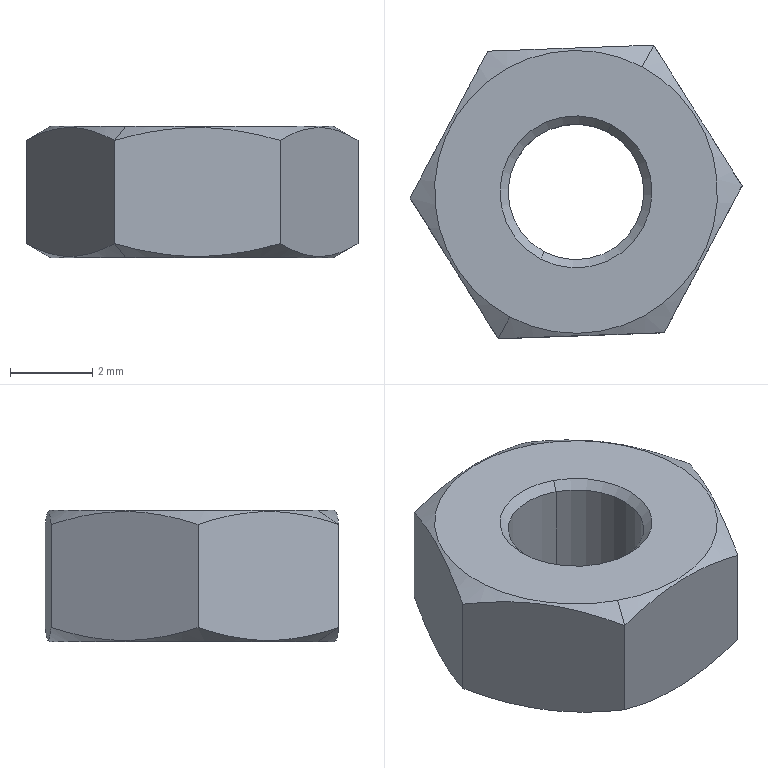Component | SolidWorks | SL010-RightStreamline-1-1_SL010-GB6171-86 M4-1-1 | 1 solid | 18 faces | box 8.08 x 7.14 x 3.2 mm | volume 107 mm3 | cone 8 | plane 8 | cylinder 2 | commonest cylinder face diameters 3.3 x2
STEP:
#1=CARTESIAN_POINT('',(10.403,-4.64,-12.324));
#2=VERTEX_POINT('',#1);
#3=CARTESIAN_POINT('',(10.463,-4.525,-12.324));
#4=VERTEX_POINT('',#3);
#5=CARTESIAN_POINT('',(10.433,-4.583,-12.324));
#6=DIRECTION('',(0.,0.,1.));
#7=DIRECTION('',(-0.4682,-0.8836,0.));
#8=AXIS2_PLACEMENT_3D('',#5,#6,#7);
#9=CIRCLE('',#8,0.06496);
#10=EDGE_CURVE('',#2,#4,#9,.T.);
#11=ORIENTED_EDGE('',*,*,#10,.F.);
#12=CARTESIAN_POINT('',(10.399,-4.647,-12.316));
#13=VERTEX_POINT('',#12);
#14=CARTESIAN_POINT('',(10.399,-4.647,-12.316));
#15=DIRECTION('',(-0.3311,-0.6248,0.7071));
#16=VECTOR('',#15,39.37);
#17=LINE('',#14,#16);
#18=EDGE_CURVE('',#2,#13,#17,.T.);
#19=ORIENTED_EDGE('',*,*,#18,.T.);
#20=CARTESIAN_POINT('',(10.467,-4.518,-12.316));
#21=VERTEX_POINT('',#20);
#22=CARTESIAN_POINT('',(10.433,-4.583,-12.316));
#23=DIRECTION('',(-0.,-0.,-1.));
#24=DIRECTION('',(-0.4682,-0.8836,0.));
#25=AXIS2_PLACEMENT_3D('',#22,#23,#24);
#26=CIRCLE('',#25,0.07283);
#27=EDGE_CURVE('',#21,#13,#26,.T.);
#28=ORIENTED_EDGE('',*,*,#27,.F.);
#29=CARTESIAN_POINT('',(10.467,-4.518,-12.316));
#30=DIRECTION('',(0.3311,0.6248,0.7071));
#31=VECTOR('',#30,39.37);
#32=LINE('',#29,#31);
#33=EDGE_CURVE('',#4,#21,#32,.T.);
#34=ORIENTED_EDGE('',*,*,#33,.F.);
#35=EDGE_LOOP('',(#11,#19,#28,#34));
#36=FACE_OUTER_BOUND('',#35,.T.);
#37=CARTESIAN_POINT('',(10.433,-4.583,-12.316));
#38=DIRECTION('',(0.,0.,1.));
#39=DIRECTION('',(0.4682,0.8836,0.));
#40=AXIS2_PLACEMENT_3D('',#37,#38,#39);
#41=CONICAL_SURFACE('',#40,0.07283,0.7854);
#42=ADVANCED_FACE('',(#36),#41,.F.);
#43=CARTESIAN_POINT('',(10.463,-4.525,-12.434));
#44=VERTEX_POINT('',#43);
#45=CARTESIAN_POINT('',(10.403,-4.64,-12.434));
#46=VERTEX_POINT('',#45);
#47=CARTESIAN_POINT('',(10.433,-4.583,-12.434));
#48=DIRECTION('',(-0.,-0.,-1.));
#49=DIRECTION('',(-0.4682,-0.8836,0.));
#50=AXIS2_PLACEMENT_3D('',#47,#48,#49);
#51=CIRCLE('',#50,0.06496);
#52=EDGE_CURVE('',#44,#46,#51,.T.);
#53=ORIENTED_EDGE('',*,*,#52,.F.);
#54=CARTESIAN_POINT('',(10.467,-4.518,-12.442));
#55=VERTEX_POINT('',#54);
#56=CARTESIAN_POINT('',(10.463,-4.525,-12.434));
#57=DIRECTION('',(0.3311,0.6248,-0.7071));
#58=VECTOR('',#57,39.37);
#59=LINE('',#56,#58);
#60=EDGE_CURVE('',#44,#55,#59,.T.);
#61=ORIENTED_EDGE('',*,*,#60,.T.);
#62=CARTESIAN_POINT('',(10.399,-4.647,-12.442));
#63=VERTEX_POINT('',#62);
#64=CARTESIAN_POINT('',(10.433,-4.583,-12.442));
#65=DIRECTION('',(0.,0.,1.));
#66=DIRECTION('',(-0.4682,-0.8836,0.));
#67=AXIS2_PLACEMENT_3D('',#64,#65,#66);
#68=CIRCLE('',#67,0.07283);
#69=EDGE_CURVE('',#63,#55,#68,.T.);
#70=ORIENTED_EDGE('',*,*,#69,.F.);
#71=CARTESIAN_POINT('',(10.403,-4.64,-12.434));
#72=DIRECTION('',(-0.3311,-0.6248,-0.7071));
#73=VECTOR('',#72,39.37);
#74=LINE('',#71,#73);
#75=EDGE_CURVE('',#46,#63,#74,.T.);
#76=ORIENTED_EDGE('',*,*,#75,.F.);
#77=EDGE_LOOP('',(#53,#61,#70,#76));
#78=FACE_OUTER_BOUND('',#77,.T.);
#79=CARTESIAN_POINT('',(10.433,-4.583,-12.434));
#80=DIRECTION('',(-0.,-0.,-1.));
#81=DIRECTION('',(-0.4682,-0.8836,0.));
#82=AXIS2_PLACEMENT_3D('',#79,#80,#81);
#83=CONICAL_SURFACE('',#82,0.06496,0.7854);
#84=ADVANCED_FACE('',(#78),#83,.F.);
#85=CARTESIAN_POINT('',(10.37,-4.703,-12.442));
#86=VERTEX_POINT('',#85);
#87=CARTESIAN_POINT('',(10.497,-4.463,-12.442));
#88=VERTEX_POINT('',#87);
#89=CARTESIAN_POINT('',(10.433,-4.583,-12.442));
#90=DIRECTION('',(0.,0.,1.));
#91=DIRECTION('',(0.4682,0.8836,0.));
#92=AXIS2_PLACEMENT_3D('',#89,#90,#91);
#93=CIRCLE('',#92,0.1355);
#94=EDGE_CURVE('',#86,#88,#93,.T.);
#95=ORIENTED_EDGE('',*,*,#94,.T.);
#96=CARTESIAN_POINT('',(10.508,-4.442,-12.429));
#97=VERTEX_POINT('',#96);
#98=CARTESIAN_POINT('',(10.497,-4.463,-12.442));
#99=DIRECTION('',(0.4055,0.7652,0.5));
#100=VECTOR('',#99,39.37);
#101=LINE('',#98,#100);
#102=EDGE_CURVE('',#88,#97,#101,.T.);
#103=ORIENTED_EDGE('',*,*,#102,.T.);
#104=CARTESIAN_POINT('',(10.592,-4.577,-12.429));
#105=VERTEX_POINT('',#104);
#106=CARTESIAN_POINT('',(10.508,-4.442,-12.429));
#107=CARTESIAN_POINT('',(10.521,-4.464,-12.436));
#108=CARTESIAN_POINT('',(10.535,-4.487,-12.441));
#109=CARTESIAN_POINT('',(10.557,-4.521,-12.441));
#110=CARTESIAN_POINT('',(10.564,-4.532,-12.44));
#111=CARTESIAN_POINT('',(10.578,-4.555,-12.436));
#112=CARTESIAN_POINT('',(10.585,-4.566,-12.432));
#113=CARTESIAN_POINT('',(10.592,-4.577,-12.429));
#114=B_SPLINE_CURVE_WITH_KNOTS('',3,(#106,#107,#108,#109,#110,#111,#112,#113),.UNSPECIFIED.,.F.,.F.,(4,2,2,4),(0.00000024,0.002041,0.003061,0.004082),.UNSPECIFIED.);
#115=EDGE_CURVE('',#97,#105,#114,.T.);
#116=ORIENTED_EDGE('',*,*,#115,.T.);
#117=CARTESIAN_POINT('',(10.518,-4.718,-12.429));
#118=VERTEX_POINT('',#117);
#119=CARTESIAN_POINT('',(10.592,-4.577,-12.429));
#120=CARTESIAN_POINT('',(10.586,-4.588,-12.432));
#121=CARTESIAN_POINT('',(10.58,-4.6,-12.436));
#122=CARTESIAN_POINT('',(10.567,-4.624,-12.44));
#123=CARTESIAN_POINT('',(10.561,-4.635,-12.441));
#124=CARTESIAN_POINT('',(10.549,-4.659,-12.441));
#125=CARTESIAN_POINT('',(10.542,-4.671,-12.44));
#126=CARTESIAN_POINT('',(10.53,-4.695,-12.436));
#127=CARTESIAN_POINT('',(10.524,-4.706,-12.432));
#128=CARTESIAN_POINT('',(10.518,-4.718,-12.429));
#129=B_SPLINE_CURVE_WITH_KNOTS('',3,(#119,#120,#121,#122,#123,#124,#125,#126,#127,#128),.UNSPECIFIED.,.F.,.F.,(4,2,2,2,4),(0.0036,0.004622,0.005645,0.006667,0.00769),.UNSPECIFIED.);
#130=EDGE_CURVE('',#105,#118,#129,.T.);
#131=ORIENTED_EDGE('',*,*,#130,.T.);
#132=CARTESIAN_POINT('',(10.359,-4.723,-12.429));
#133=VERTEX_POINT('',#132);
#134=CARTESIAN_POINT('',(10.518,-4.718,-12.429));
#135=CARTESIAN_POINT('',(10.492,-4.719,-12.436));
#136=CARTESIAN_POINT('',(10.465,-4.72,-12.441));
#137=CARTESIAN_POINT('',(10.425,-4.721,-12.441));
#138=CARTESIAN_POINT('',(10.411,-4.722,-12.44));
#139=CARTESIAN_POINT('',(10.385,-4.722,-12.436));
#140=CARTESIAN_POINT('',(10.372,-4.723,-12.432));
#141=CARTESIAN_POINT('',(10.359,-4.723,-12.429));
#142=B_SPLINE_CURVE_WITH_KNOTS('',3,(#134,#135,#136,#137,#138,#139,#140,#141),.UNSPECIFIED.,.F.,.F.,(4,2,2,4),(0.00000024,0.002041,0.003061,0.004082),.UNSPECIFIED.);
#143=EDGE_CURVE('',#118,#133,#142,.T.);
#144=ORIENTED_EDGE('',*,*,#143,.T.);
#145=CARTESIAN_POINT('',(10.37,-4.703,-12.442));
#146=DIRECTION('',(-0.4055,-0.7652,0.5));
#147=VECTOR('',#146,39.37);
#148=LINE('',#145,#147);
#149=EDGE_CURVE('',#86,#133,#148,.T.);
#150=ORIENTED_EDGE('',*,*,#149,.F.);
#151=EDGE_LOOP('',(#95,#103,#116,#131,#144,#150));
#152=FACE_OUTER_BOUND('',#151,.T.);
#153=CARTESIAN_POINT('',(10.433,-4.583,-12.442));
#154=DIRECTION('',(0.,0.,1.));
#155=DIRECTION('',(-0.4682,-0.8836,0.));
#156=AXIS2_PLACEMENT_3D('',#153,#154,#155);
#157=CONICAL_SURFACE('',#156,0.1355,1.047);
#158=ADVANCED_FACE('',(#152),#157,.T.);
#159=CARTESIAN_POINT('',(10.497,-4.463,-12.316));
#160=VERTEX_POINT('',#159);
#161=CARTESIAN_POINT('',(10.37,-4.703,-12.316));
#162=VERTEX_POINT('',#161);
#163=CARTESIAN_POINT('',(10.433,-4.583,-12.316));
#164=DIRECTION('',(0.,0.,1.));
#165=DIRECTION('',(0.4682,0.8836,0.));
#166=AXIS2_PLACEMENT_3D('',#163,#164,#165);
#167=CIRCLE('',#166,0.1355);
#168=EDGE_CURVE('',#160,#162,#167,.T.);
#169=ORIENTED_EDGE('',*,*,#168,.F.);
#170=CARTESIAN_POINT('',(10.508,-4.442,-12.33));
#171=VERTEX_POINT('',#170);
#172=CARTESIAN_POINT('',(10.497,-4.463,-12.316));
#173=DIRECTION('',(0.4055,0.7652,-0.5));
#174=VECTOR('',#173,39.37);
#175=LINE('',#172,#174);
#176=EDGE_CURVE('',#160,#171,#175,.T.);
#177=ORIENTED_EDGE('',*,*,#176,.T.);
#178=CARTESIAN_POINT('',(10.349,-4.448,-12.33));
#179=VERTEX_POINT('',#178);
#180=CARTESIAN_POINT('',(10.508,-4.442,-12.33));
#181=CARTESIAN_POINT('',(10.482,-4.443,-12.322));
#182=CARTESIAN_POINT('',(10.455,-4.444,-12.318));
#183=CARTESIAN_POINT('',(10.415,-4.446,-12.318));
#184=CARTESIAN_POINT('',(10.401,-4.446,-12.319));
#185=CARTESIAN_POINT('',(10.375,-4.447,-12.323));
#186=CARTESIAN_POINT('',(10.362,-4.448,-12.326));
#187=CARTESIAN_POINT('',(10.349,-4.448,-12.33));
#188=B_SPLINE_CURVE_WITH_KNOTS('',3,(#180,#181,#182,#183,#184,#185,#186,#187),.UNSPECIFIED.,.F.,.F.,(4,2,2,4),(0.00000024,0.002041,0.003061,0.004082),.UNSPECIFIED.);
#189=EDGE_CURVE('',#171,#179,#188,.T.);
#190=ORIENTED_EDGE('',*,*,#189,.T.);
#191=CARTESIAN_POINT('',(10.274,-4.589,-12.33));
#192=VERTEX_POINT('',#191);
#193=CARTESIAN_POINT('',(10.349,-4.448,-12.33));
#194=CARTESIAN_POINT('',(10.342,-4.459,-12.326));
#195=CARTESIAN_POINT('',(10.336,-4.471,-12.323));
#196=CARTESIAN_POINT('',(10.324,-4.495,-12.319));
#197=CARTESIAN_POINT('',(10.318,-4.506,-12.318));
#198=CARTESIAN_POINT('',(10.305,-4.53,-12.318));
#199=CARTESIAN_POINT('',(10.299,-4.542,-12.319));
#200=CARTESIAN_POINT('',(10.286,-4.566,-12.323));
#201=CARTESIAN_POINT('',(10.28,-4.577,-12.326));
#202=CARTESIAN_POINT('',(10.274,-4.589,-12.33));
#203=B_SPLINE_CURVE_WITH_KNOTS('',3,(#193,#194,#195,#196,#197,#198,#199,#200,#201,#202),.UNSPECIFIED.,.F.,.F.,(4,2,2,2,4),(0.0036,0.004622,0.005645,0.006667,0.00769),.UNSPECIFIED.);
#204=EDGE_CURVE('',#179,#192,#203,.T.);
#205=ORIENTED_EDGE('',*,*,#204,.T.);
#206=CARTESIAN_POINT('',(10.359,-4.723,-12.33));
#207=VERTEX_POINT('',#206);
#208=CARTESIAN_POINT('',(10.274,-4.589,-12.33));
#209=CARTESIAN_POINT('',(10.288,-4.611,-12.322));
#210=CARTESIAN_POINT('',(10.302,-4.633,-12.318));
#211=CARTESIAN_POINT('',(10.323,-4.667,-12.318));
#212=CARTESIAN_POINT('',(10.331,-4.679,-12.319));
#213=CARTESIAN_POINT('',(10.345,-4.701,-12.323));
#214=CARTESIAN_POINT('',(10.352,-4.712,-12.326));
#215=CARTESIAN_POINT('',(10.359,-4.723,-12.33));
#216=B_SPLINE_CURVE_WITH_KNOTS('',3,(#208,#209,#210,#211,#212,#213,#214,#215),.UNSPECIFIED.,.F.,.F.,(4,2,2,4),(0.00000024,0.002041,0.003061,0.004082),.UNSPECIFIED.);
#217=EDGE_CURVE('',#192,#207,#216,.T.);
#218=ORIENTED_EDGE('',*,*,#217,.T.);
#219=CARTESIAN_POINT('',(10.37,-4.703,-12.316));
#220=DIRECTION('',(-0.4055,-0.7652,-0.5));
#221=VECTOR('',#220,39.37);
#222=LINE('',#219,#221);
#223=EDGE_CURVE('',#162,#207,#222,.T.);
#224=ORIENTED_EDGE('',*,*,#223,.F.);
#225=EDGE_LOOP('',(#169,#177,#190,#205,#218,#224));
#226=FACE_OUTER_BOUND('',#225,.T.);
#227=CARTESIAN_POINT('',(10.433,-4.583,-12.316));
#228=DIRECTION('',(-0.,-0.,-1.));
#229=DIRECTION('',(-0.4682,-0.8836,0.));
#230=AXIS2_PLACEMENT_3D('',#227,#228,#229);
#231=CONICAL_SURFACE('',#230,0.1355,1.047);
#232=ADVANCED_FACE('',(#226),#231,.T.);
#233=ORIENTED_EDGE('',*,*,#10,.T.);
#234=CARTESIAN_POINT('',(10.463,-4.525,-12.442));
#235=DIRECTION('',(-0.,-0.,-1.));
#236=VECTOR('',#235,39.37);
#237=LINE('',#234,#236);
#238=EDGE_CURVE('',#4,#44,#237,.T.);
#239=ORIENTED_EDGE('',*,*,#238,.T.);
#240=ORIENTED_EDGE('',*,*,#52,.T.);
#241=CARTESIAN_POINT('',(10.403,-4.64,-12.442));
#242=DIRECTION('',(-0.,-0.,-1.));
#243=VECTOR('',#242,39.37);
#244=LINE('',#241,#243);
#245=EDGE_CURVE('',#2,#46,#244,.T.);
#246=ORIENTED_EDGE('',*,*,#245,.F.);
#247=EDGE_LOOP('',(#233,#239,#240,#246));
#248=FACE_OUTER_BOUND('',#247,.T.);
#249=CARTESIAN_POINT('',(10.433,-4.583,-12.442));
#250=DIRECTION('',(-0.,-0.,-1.));
#251=DIRECTION('',(-0.4682,-0.8836,0.));
#252=AXIS2_PLACEMENT_3D('',#249,#250,#251);
#253=CYLINDRICAL_SURFACE('',#252,0.06496);
#254=ADVANCED_FACE('',(#248),#253,.F.);
#255=ORIENTED_EDGE('',*,*,#143,.F.);
#256=CARTESIAN_POINT('',(10.518,-4.718,-12.33));
#257=VERTEX_POINT('',#256);
#258=CARTESIAN_POINT('',(10.518,-4.718,-12.442));
#259=DIRECTION('',(0.,0.,1.));
#260=VECTOR('',#259,39.37);
#261=LINE('',#258,#260);
#262=EDGE_CURVE('',#118,#257,#261,.T.);
#263=ORIENTED_EDGE('',*,*,#262,.T.);
#264=CARTESIAN_POINT('',(10.359,-4.723,-12.33));
#265=CARTESIAN_POINT('',(10.385,-4.722,-12.322));
#266=CARTESIAN_POINT('',(10.411,-4.722,-12.318));
#267=CARTESIAN_POINT('',(10.451,-4.72,-12.318));
#268=CARTESIAN_POINT('',(10.465,-4.72,-12.319));
#269=CARTESIAN_POINT('',(10.491,-4.719,-12.323));
#270=CARTESIAN_POINT('',(10.505,-4.718,-12.326));
#271=CARTESIAN_POINT('',(10.518,-4.718,-12.33));
#272=B_SPLINE_CURVE_WITH_KNOTS('',3,(#264,#265,#266,#267,#268,#269,#270,#271),.UNSPECIFIED.,.F.,.F.,(4,2,2,4),(0.00000024,0.002041,0.003061,0.004082),.UNSPECIFIED.);
#273=EDGE_CURVE('',#207,#257,#272,.T.);
#274=ORIENTED_EDGE('',*,*,#273,.F.);
#275=CARTESIAN_POINT('',(10.359,-4.723,-12.442));
#276=DIRECTION('',(0.,0.,1.));
#277=VECTOR('',#276,39.37);
#278=LINE('',#275,#277);
#279=EDGE_CURVE('',#133,#207,#278,.T.);
#280=ORIENTED_EDGE('',*,*,#279,.F.);
#281=EDGE_LOOP('',(#255,#263,#274,#280));
#282=FACE_OUTER_BOUND('',#281,.T.);
#283=CARTESIAN_POINT('',(10.518,-4.718,-12.442));
#284=DIRECTION('',(-0.03636,0.9993,-0.));
#285=DIRECTION('',(0.9993,0.03636,-0.));
#286=AXIS2_PLACEMENT_3D('',#283,#284,#285);
#287=PLANE('',#286);
#288=ADVANCED_FACE('',(#282),#287,.F.);
#289=CARTESIAN_POINT('',(10.274,-4.589,-12.429));
#290=VERTEX_POINT('',#289);
#291=CARTESIAN_POINT('',(10.359,-4.723,-12.429));
#292=CARTESIAN_POINT('',(10.345,-4.701,-12.436));
#293=CARTESIAN_POINT('',(10.331,-4.679,-12.441));
#294=CARTESIAN_POINT('',(10.309,-4.645,-12.441));
#295=CARTESIAN_POINT('',(10.302,-4.633,-12.44));
#296=CARTESIAN_POINT('',(10.288,-4.611,-12.436));
#297=CARTESIAN_POINT('',(10.281,-4.6,-12.432));
#298=CARTESIAN_POINT('',(10.274,-4.589,-12.429));
#299=B_SPLINE_CURVE_WITH_KNOTS('',3,(#291,#292,#293,#294,#295,#296,#297,#298),.UNSPECIFIED.,.F.,.F.,(4,2,2,4),(0.00000024,0.002041,0.003061,0.004082),.UNSPECIFIED.);
#300=EDGE_CURVE('',#133,#290,#299,.T.);
#301=ORIENTED_EDGE('',*,*,#300,.F.);
#302=ORIENTED_EDGE('',*,*,#279,.T.);
#303=ORIENTED_EDGE('',*,*,#217,.F.);
#304=CARTESIAN_POINT('',(10.274,-4.589,-12.442));
#305=DIRECTION('',(0.,0.,1.));
#306=VECTOR('',#305,39.37);
#307=LINE('',#304,#306);
#308=EDGE_CURVE('',#290,#192,#307,.T.);
#309=ORIENTED_EDGE('',*,*,#308,.F.);
#310=EDGE_LOOP('',(#301,#302,#303,#309));
#311=FACE_OUTER_BOUND('',#310,.T.);
#312=CARTESIAN_POINT('',(10.359,-4.723,-12.442));
#313=DIRECTION('',(0.8473,0.5312,-0.));
#314=DIRECTION('',(0.5312,-0.8473,0.));
#315=AXIS2_PLACEMENT_3D('',#312,#313,#314);
#316=PLANE('',#315);
#317=ADVANCED_FACE('',(#311),#316,.F.);
#318=CARTESIAN_POINT('',(10.349,-4.448,-12.429));
#319=VERTEX_POINT('',#318);
#320=CARTESIAN_POINT('',(10.274,-4.589,-12.429));
#321=CARTESIAN_POINT('',(10.28,-4.577,-12.432));
#322=CARTESIAN_POINT('',(10.286,-4.566,-12.436));
#323=CARTESIAN_POINT('',(10.299,-4.542,-12.44));
#324=CARTESIAN_POINT('',(10.305,-4.53,-12.441));
#325=CARTESIAN_POINT('',(10.318,-4.506,-12.441));
#326=CARTESIAN_POINT('',(10.324,-4.495,-12.44));
#327=CARTESIAN_POINT('',(10.336,-4.471,-12.436));
#328=CARTESIAN_POINT('',(10.342,-4.459,-12.432));
#329=CARTESIAN_POINT('',(10.349,-4.448,-12.429));
#330=B_SPLINE_CURVE_WITH_KNOTS('',3,(#320,#321,#322,#323,#324,#325,#326,#327,#328,#329),.UNSPECIFIED.,.F.,.F.,(4,2,2,2,4),(0.001487,0.002507,0.003526,0.004546,0.005566),.UNSPECIFIED.);
#331=EDGE_CURVE('',#290,#319,#330,.T.);
#332=ORIENTED_EDGE('',*,*,#331,.F.);
#333=ORIENTED_EDGE('',*,*,#308,.T.);
#334=ORIENTED_EDGE('',*,*,#204,.F.);
#335=CARTESIAN_POINT('',(10.349,-4.448,-12.442));
#336=DIRECTION('',(0.,0.,1.));
#337=VECTOR('',#336,39.37);
#338=LINE('',#335,#337);
#339=EDGE_CURVE('',#319,#179,#338,.T.);
#340=ORIENTED_EDGE('',*,*,#339,.F.);
#341=EDGE_LOOP('',(#332,#333,#334,#340));
#342=FACE_OUTER_BOUND('',#341,.T.);
#343=CARTESIAN_POINT('',(10.274,-4.589,-12.442));
#344=DIRECTION('',(0.8836,-0.4682,0.));
#345=DIRECTION('',(0.,0.,1.));
#346=AXIS2_PLACEMENT_3D('',#343,#344,#345);
#347=PLANE('',#346);
#348=ADVANCED_FACE('',(#342),#347,.F.);
#349=CARTESIAN_POINT('',(10.349,-4.448,-12.429));
#350=CARTESIAN_POINT('',(10.375,-4.447,-12.436));
#351=CARTESIAN_POINT('',(10.401,-4.446,-12.441));
#352=CARTESIAN_POINT('',(10.441,-4.445,-12.441));
#353=CARTESIAN_POINT('',(10.455,-4.444,-12.44));
#354=CARTESIAN_POINT('',(10.481,-4.443,-12.436));
#355=CARTESIAN_POINT('',(10.495,-4.443,-12.432));
#356=CARTESIAN_POINT('',(10.508,-4.442,-12.429));
#357=B_SPLINE_CURVE_WITH_KNOTS('',3,(#349,#350,#351,#352,#353,#354,#355,#356),.UNSPECIFIED.,.F.,.F.,(4,2,2,4),(0.00000024,0.002041,0.003061,0.004082),.UNSPECIFIED.);
#358=EDGE_CURVE('',#319,#97,#357,.T.);
#359=ORIENTED_EDGE('',*,*,#358,.F.);
#360=ORIENTED_EDGE('',*,*,#339,.T.);
#361=ORIENTED_EDGE('',*,*,#189,.F.);
#362=CARTESIAN_POINT('',(10.508,-4.442,-12.442));
#363=DIRECTION('',(0.,0.,1.));
#364=VECTOR('',#363,39.37);
#365=LINE('',#362,#364);
#366=EDGE_CURVE('',#97,#171,#365,.T.);
#367=ORIENTED_EDGE('',*,*,#366,.F.);
#368=EDGE_LOOP('',(#359,#360,#361,#367));
#369=FACE_OUTER_BOUND('',#368,.T.);
#370=CARTESIAN_POINT('',(10.349,-4.448,-12.442));
#371=DIRECTION('',(0.03636,-0.9993,0.));
#372=DIRECTION('',(-0.9993,-0.03636,0.));
#373=AXIS2_PLACEMENT_3D('',#370,#371,#372);
#374=PLANE('',#373);
#375=ADVANCED_FACE('',(#369),#374,.F.);
#376=ORIENTED_EDGE('',*,*,#115,.F.);
#377=ORIENTED_EDGE('',*,*,#366,.T.);
#378=CARTESIAN_POINT('',(10.592,-4.577,-12.33));
#379=VERTEX_POINT('',#378);
#380=CARTESIAN_POINT('',(10.592,-4.577,-12.33));
#381=CARTESIAN_POINT('',(10.578,-4.555,-12.322));
#382=CARTESIAN_POINT('',(10.564,-4.533,-12.318));
#383=CARTESIAN_POINT('',(10.543,-4.498,-12.318));
#384=CARTESIAN_POINT('',(10.536,-4.487,-12.319));
#385=CARTESIAN_POINT('',(10.521,-4.464,-12.323));
#386=CARTESIAN_POINT('',(10.514,-4.453,-12.326));
#387=CARTESIAN_POINT('',(10.508,-4.442,-12.33));
#388=B_SPLINE_CURVE_WITH_KNOTS('',3,(#380,#381,#382,#383,#384,#385,#386,#387),.UNSPECIFIED.,.F.,.F.,(4,2,2,4),(0.00000024,0.002041,0.003061,0.004082),.UNSPECIFIED.);
#389=EDGE_CURVE('',#379,#171,#388,.T.);
#390=ORIENTED_EDGE('',*,*,#389,.F.);
#391=CARTESIAN_POINT('',(10.592,-4.577,-12.442));
#392=DIRECTION('',(0.,0.,1.));
#393=VECTOR('',#392,39.37);
#394=LINE('',#391,#393);
#395=EDGE_CURVE('',#105,#379,#394,.T.);
#396=ORIENTED_EDGE('',*,*,#395,.F.);
#397=EDGE_LOOP('',(#376,#377,#390,#396));
#398=FACE_OUTER_BOUND('',#397,.T.);
#399=CARTESIAN_POINT('',(10.508,-4.442,-12.442));
#400=DIRECTION('',(-0.8473,-0.5312,0.));
#401=DIRECTION('',(-0.5312,0.8473,-0.));
#402=AXIS2_PLACEMENT_3D('',#399,#400,#401);
#403=PLANE('',#402);
#404=ADVANCED_FACE('',(#398),#403,.F.);
#405=ORIENTED_EDGE('',*,*,#130,.F.);
#406=ORIENTED_EDGE('',*,*,#395,.T.);
#407=CARTESIAN_POINT('',(10.518,-4.718,-12.33));
#408=CARTESIAN_POINT('',(10.524,-4.706,-12.326));
#409=CARTESIAN_POINT('',(10.53,-4.695,-12.323));
#410=CARTESIAN_POINT('',(10.542,-4.671,-12.319));
#411=CARTESIAN_POINT('',(10.549,-4.659,-12.318));
#412=CARTESIAN_POINT('',(10.561,-4.635,-12.318));
#413=CARTESIAN_POINT('',(10.567,-4.624,-12.319));
#414=CARTESIAN_POINT('',(10.58,-4.6,-12.323));
#415=CARTESIAN_POINT('',(10.586,-4.588,-12.326));
#416=CARTESIAN_POINT('',(10.592,-4.577,-12.33));
#417=B_SPLINE_CURVE_WITH_KNOTS('',3,(#407,#408,#409,#410,#411,#412,#413,#414,#415,#416),.UNSPECIFIED.,.F.,.F.,(4,2,2,2,4),(0.001487,0.002507,0.003526,0.004546,0.005566),.UNSPECIFIED.);
#418=EDGE_CURVE('',#257,#379,#417,.T.);
#419=ORIENTED_EDGE('',*,*,#418,.F.);
#420=ORIENTED_EDGE('',*,*,#262,.F.);
#421=EDGE_LOOP('',(#405,#406,#419,#420));
#422=FACE_OUTER_BOUND('',#421,.T.);
#423=CARTESIAN_POINT('',(10.592,-4.577,-12.442));
#424=DIRECTION('',(-0.8836,0.4682,-0.));
#425=DIRECTION('',(-0.,-0.,-1.));
#426=AXIS2_PLACEMENT_3D('',#423,#424,#425);
#427=PLANE('',#426);
#428=ADVANCED_FACE('',(#422),#427,.F.);
#429=ORIENTED_EDGE('',*,*,#69,.T.);
#430=CARTESIAN_POINT('',(10.433,-4.583,-12.442));
#431=DIRECTION('',(0.,0.,1.));
#432=DIRECTION('',(-0.4682,-0.8836,0.));
#433=AXIS2_PLACEMENT_3D('',#430,#431,#432);
#434=CIRCLE('',#433,0.07283);
#435=EDGE_CURVE('',#55,#63,#434,.T.);
#436=ORIENTED_EDGE('',*,*,#435,.T.);
#437=EDGE_LOOP('',(#429,#436));
#438=FACE_BOUND('',#437,.T.);
#439=ORIENTED_EDGE('',*,*,#94,.F.);
#440=CARTESIAN_POINT('',(10.433,-4.583,-12.442));
#441=DIRECTION('',(0.,0.,1.));
#442=DIRECTION('',(0.4682,0.8836,0.));
#443=AXIS2_PLACEMENT_3D('',#440,#441,#442);
#444=CIRCLE('',#443,0.1355);
#445=EDGE_CURVE('',#88,#86,#444,.T.);
#446=ORIENTED_EDGE('',*,*,#445,.F.);
#447=EDGE_LOOP('',(#439,#446));
#448=FACE_OUTER_BOUND('',#447,.T.);
#449=CARTESIAN_POINT('',(10.359,-4.723,-12.442));
#450=DIRECTION('',(-0.,-0.,-1.));
#451=DIRECTION('',(-0.4682,-0.8836,0.));
#452=AXIS2_PLACEMENT_3D('',#449,#450,#451);
#453=PLANE('',#452);
#454=ADVANCED_FACE('',(#438,#448),#453,.T.);
#455=ORIENTED_EDGE('',*,*,#27,.T.);
#456=CARTESIAN_POINT('',(10.433,-4.583,-12.316));
#457=DIRECTION('',(-0.,-0.,-1.));
#458=DIRECTION('',(-0.4682,-0.8836,0.));
#459=AXIS2_PLACEMENT_3D('',#456,#457,#458);
#460=CIRCLE('',#459,0.07283);
#461=EDGE_CURVE('',#13,#21,#460,.T.);
#462=ORIENTED_EDGE('',*,*,#461,.T.);
#463=EDGE_LOOP('',(#455,#462));
#464=FACE_BOUND('',#463,.T.);
#465=CARTESIAN_POINT('',(10.433,-4.583,-12.316));
#466=DIRECTION('',(0.,0.,1.));
#467=DIRECTION('',(0.4682,0.8836,0.));
#468=AXIS2_PLACEMENT_3D('',#465,#466,#467);
#469=CIRCLE('',#468,0.1355);
#470=EDGE_CURVE('',#162,#160,#469,.T.);
#471=ORIENTED_EDGE('',*,*,#470,.T.);
#472=ORIENTED_EDGE('',*,*,#168,.T.);
#473=EDGE_LOOP('',(#471,#472));
#474=FACE_OUTER_BOUND('',#473,.T.);
#475=CARTESIAN_POINT('',(10.359,-4.723,-12.316));
#476=DIRECTION('',(-0.,-0.,-1.));
#477=DIRECTION('',(-0.4682,-0.8836,0.));
#478=AXIS2_PLACEMENT_3D('',#475,#476,#477);
#479=PLANE('',#478);
#480=ADVANCED_FACE('',(#464,#474),#479,.F.);
#481=ORIENTED_EDGE('',*,*,#238,.F.);
#482=CARTESIAN_POINT('',(10.433,-4.583,-12.324));
#483=DIRECTION('',(0.,0.,1.));
#484=DIRECTION('',(-0.4682,-0.8836,0.));
#485=AXIS2_PLACEMENT_3D('',#482,#483,#484);
#486=CIRCLE('',#485,0.06496);
#487=EDGE_CURVE('',#4,#2,#486,.T.);
#488=ORIENTED_EDGE('',*,*,#487,.T.);
#489=ORIENTED_EDGE('',*,*,#245,.T.);
#490=CARTESIAN_POINT('',(10.433,-4.583,-12.434));
#491=DIRECTION('',(-0.,-0.,-1.));
#492=DIRECTION('',(-0.4682,-0.8836,0.));
#493=AXIS2_PLACEMENT_3D('',#490,#491,#492);
#494=CIRCLE('',#493,0.06496);
#495=EDGE_CURVE('',#46,#44,#494,.T.);
#496=ORIENTED_EDGE('',*,*,#495,.T.);
#497=EDGE_LOOP('',(#481,#488,#489,#496));
#498=FACE_OUTER_BOUND('',#497,.T.);
#499=CARTESIAN_POINT('',(10.433,-4.583,-12.442));
#500=DIRECTION('',(-0.,-0.,-1.));
#501=DIRECTION('',(-0.4682,-0.8836,0.));
#502=AXIS2_PLACEMENT_3D('',#499,#500,#501);
#503=CYLINDRICAL_SURFACE('',#502,0.06496);
#504=ADVANCED_FACE('',(#498),#503,.F.);
#505=ORIENTED_EDGE('',*,*,#176,.F.);
#506=ORIENTED_EDGE('',*,*,#470,.F.);
#507=ORIENTED_EDGE('',*,*,#223,.T.);
#508=ORIENTED_EDGE('',*,*,#273,.T.);
#509=ORIENTED_EDGE('',*,*,#418,.T.);
#510=ORIENTED_EDGE('',*,*,#389,.T.);
#511=EDGE_LOOP('',(#505,#506,#507,#508,#509,#510));
#512=FACE_OUTER_BOUND('',#511,.T.);
#513=CARTESIAN_POINT('',(10.433,-4.583,-12.316));
#514=DIRECTION('',(-0.,-0.,-1.));
#515=DIRECTION('',(-0.4682,-0.8836,0.));
#516=AXIS2_PLACEMENT_3D('',#513,#514,#515);
#517=CONICAL_SURFACE('',#516,0.1355,1.047);
#518=ADVANCED_FACE('',(#512),#517,.T.);
#519=ORIENTED_EDGE('',*,*,#102,.F.);
#520=ORIENTED_EDGE('',*,*,#445,.T.);
#521=ORIENTED_EDGE('',*,*,#149,.T.);
#522=ORIENTED_EDGE('',*,*,#300,.T.);
#523=ORIENTED_EDGE('',*,*,#331,.T.);
#524=ORIENTED_EDGE('',*,*,#358,.T.);
#525=EDGE_LOOP('',(#519,#520,#521,#522,#523,#524));
#526=FACE_OUTER_BOUND('',#525,.T.);
#527=CARTESIAN_POINT('',(10.433,-4.583,-12.442));
#528=DIRECTION('',(0.,0.,1.));
#529=DIRECTION('',(-0.4682,-0.8836,0.));
#530=AXIS2_PLACEMENT_3D('',#527,#528,#529);
#531=CONICAL_SURFACE('',#530,0.1355,1.047);
#532=ADVANCED_FACE('',(#526),#531,.T.);
#533=ORIENTED_EDGE('',*,*,#60,.F.);
#534=ORIENTED_EDGE('',*,*,#495,.F.);
#535=ORIENTED_EDGE('',*,*,#75,.T.);
#536=ORIENTED_EDGE('',*,*,#435,.F.);
#537=EDGE_LOOP('',(#533,#534,#535,#536));
#538=FACE_OUTER_BOUND('',#537,.T.);
#539=CARTESIAN_POINT('',(10.433,-4.583,-12.434));
#540=DIRECTION('',(-0.,-0.,-1.));
#541=DIRECTION('',(-0.4682,-0.8836,0.));
#542=AXIS2_PLACEMENT_3D('',#539,#540,#541);
#543=CONICAL_SURFACE('',#542,0.06496,0.7854);
#544=ADVANCED_FACE('',(#538),#543,.F.);
#545=ORIENTED_EDGE('',*,*,#18,.F.);
#546=ORIENTED_EDGE('',*,*,#487,.F.);
#547=ORIENTED_EDGE('',*,*,#33,.T.);
#548=ORIENTED_EDGE('',*,*,#461,.F.);
#549=EDGE_LOOP('',(#545,#546,#547,#548));
#550=FACE_OUTER_BOUND('',#549,.T.);
#551=CARTESIAN_POINT('',(10.433,-4.583,-12.316));
#552=DIRECTION('',(0.,0.,1.));
#553=DIRECTION('',(0.4682,0.8836,0.));
#554=AXIS2_PLACEMENT_3D('',#551,#552,#553);
#555=CONICAL_SURFACE('',#554,0.07283,0.7854);
#556=ADVANCED_FACE('',(#550),#555,.F.);
#557=CLOSED_SHELL('',(#42,#84,#158,#232,#254,#288,#317,#348,#375,#404,#428,#454,#480,#504,#518,#532,#544,#556));
#558=MANIFOLD_SOLID_BREP('',#557);
#559=CARTESIAN_POINT('',(0.,0.,0.));
#560=DIRECTION('',(0.,0.,1.));
#561=DIRECTION('',(1.,0.,0.));
#562=AXIS2_PLACEMENT_3D('',#559,#560,#561);
#563=(LENGTH_UNIT()NAMED_UNIT(*)SI_UNIT($,.METRE.));
#564=LENGTH_MEASURE_WITH_UNIT(LENGTH_MEASURE(0.0254),#563);
#565=DIMENSIONAL_EXPONENTS(1.,0.,0.,0.,0.,0.,0.);
#566=(CONVERSION_BASED_UNIT('',#564)LENGTH_UNIT()NAMED_UNIT(#565));
#567=UNCERTAINTY_MEASURE_WITH_UNIT(LENGTH_MEASURE(0.00001),#566,'','');
#568=(NAMED_UNIT(*)PLANE_ANGLE_UNIT()SI_UNIT($,.RADIAN.));
#569=(NAMED_UNIT(*)SI_UNIT($,.STERADIAN.)SOLID_ANGLE_UNIT());
#570=(GEOMETRIC_REPRESENTATION_CONTEXT(3)GLOBAL_UNCERTAINTY_ASSIGNED_CONTEXT((#567))GLOBAL_UNIT_ASSIGNED_CONTEXT((#566,#568,#569))REPRESENTATION_CONTEXT('',''));
#571=ADVANCED_BREP_SHAPE_REPRESENTATION('',(#558,#562),#570);
#572=COLOUR_RGB('',0.7922,0.8196,0.9333);
#573=FILL_AREA_STYLE_COLOUR('',#572);
#574=FILL_AREA_STYLE('',(#573));
#575=SURFACE_STYLE_FILL_AREA(#574);
#576=SURFACE_SIDE_STYLE('',(#575));
#577=SURFACE_STYLE_USAGE(.BOTH.,#576);
#578=PRESENTATION_STYLE_ASSIGNMENT((#577));
#579=STYLED_ITEM('',(#578),#558);
#580=PRESENTATION_LAYER_ASSIGNMENT('','',(#579));
#581=(LENGTH_UNIT()NAMED_UNIT(*)SI_UNIT($,.METRE.));
#582=LENGTH_MEASURE_WITH_UNIT(LENGTH_MEASURE(0.0254),#581);
#583=DIMENSIONAL_EXPONENTS(1.,0.,0.,0.,0.,0.,0.);
#584=(CONVERSION_BASED_UNIT('',#582)LENGTH_UNIT()NAMED_UNIT(#583));
#585=UNCERTAINTY_MEASURE_WITH_UNIT(LENGTH_MEASURE(0.00001),#584,'','');
#586=(NAMED_UNIT(*)PLANE_ANGLE_UNIT()SI_UNIT($,.RADIAN.));
#587=(NAMED_UNIT(*)SI_UNIT($,.STERADIAN.)SOLID_ANGLE_UNIT());
#588=(GEOMETRIC_REPRESENTATION_CONTEXT(3)GLOBAL_UNCERTAINTY_ASSIGNED_CONTEXT((#585))GLOBAL_UNIT_ASSIGNED_CONTEXT((#584,#586,#587))REPRESENTATION_CONTEXT('',''));
#589=MECHANICAL_DESIGN_GEOMETRIC_PRESENTATION_REPRESENTATION('',(#579),#588);